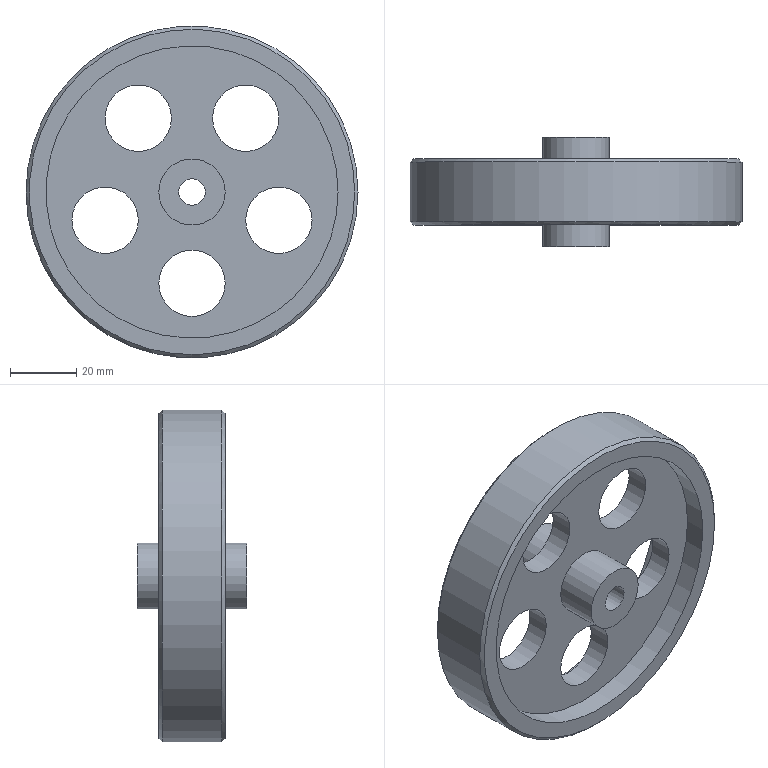Component | NX | FLYWHEEL | 1 solid | 19 faces | volume 73214 mm3 | cylinder 11 | plane 6 | cone 2 | commonest cylinder face diameters 20 x7 88 x2 100 x1 8 x1